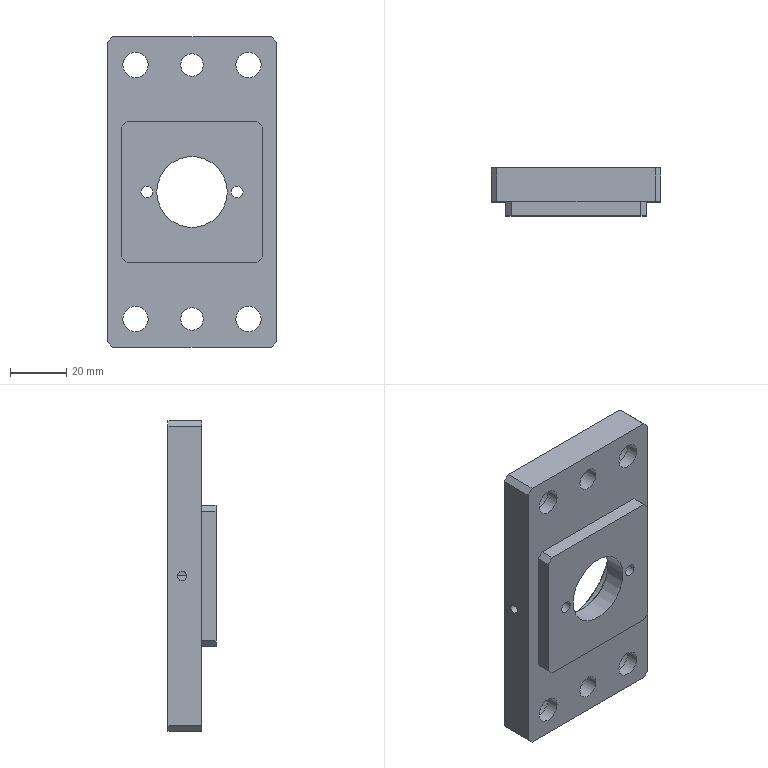Component | SolidWorks | 300-02-1 | 1 solid | 114 faces | box 60 x 17 x 110 mm | volume 65342 mm3 | plane 50 | cylinder 30 | spline 30 | cone 4 | commonest cylinder face diameters 15 x8 9 x8 8 x4 4.2 x4 3.3 x2 45 x2 25 x2 | material Cr12MoV
build123d program:
from build123d import *

# Parameters (mm, degrees)
SKETCH1_W                                          = 110
SKETCH1_H                                          = 60
BOSS_EXTRUDE1_DEPTH                                = 12
CHAMFER1_SIZE                                      = 2
SKETCH9_W                                          = 50
SKETCH9_H                                          = 50
BOSS_EXTRUDE2_DEPTH                                = 5
SKETCH2_R                                          = 12.5
CUT_EXTRUDE1_DEPTH                                 = 65.915
SKETCH5_R                                          = 22.5
CUT_EXTRUDE2_DEPTH                                 = 9
M5_TAPPED_HOLE1_D                                  = 4.2
CHAMFER2_SIZE                                      = 2
HOLE_SIZE_ACCORDING_TO_TYPE_OF_HEXAGON_D           = 9
HOLE_SIZE_ACCORDING_TO_TYPE_OF_HEXAGON_CBORE_D     = 15
HOLE_SIZE_ACCORDING_TO_TYPE_OF_HEXAGON_CBORE_DEPTH = 7.5
SIZE_MM_DOWEL_PIN_HOLE1_D                          = 8
CHAMFER3_SIZE                                      = 0.5
CUT_EXTRUDE3_DEPTH                                 = 0.2
M4_TAPPED_HOLE1_REACH                              = 84.274
M4_TAPPED_HOLE1_BORE_R                             = 1.65


with BuildPart() as part:
    # Sketch1 → Boss-Extrude1 (new body)
    with BuildSketch(Plane(origin=(0, 0, 0), x_dir=(1, 0, 0), z_dir=(0, 1, 0))):
        Rectangle(SKETCH1_W, SKETCH1_H)
    extrude(amount=BOSS_EXTRUDE1_DEPTH)

    # Chamfer1
    chamfer1_edges = [part.edges().sort_by_distance(p)[0] for p in [
        (-55, 6, -30),
        (55, 6, -30),
        (55, 6, 30),
        (-55, 6, 30),
    ]]
    chamfer(chamfer1_edges, length=CHAMFER1_SIZE)

    # Sketch9 → Boss-Extrude2 (add)
    with BuildSketch(Plane.XZ):
        Rectangle(SKETCH9_W, SKETCH9_H)
    extrude(amount=BOSS_EXTRUDE2_DEPTH)

    # Sketch2 → Cut-Extrude1 (cut, through all)
    with BuildSketch(Plane(origin=(0, 12, 0), x_dir=(1, 0, 0), z_dir=(0, 1, 0))):
        with Locations(Location((0, 0, 0), (0, 0, 270))):
            Circle(SKETCH2_R)
    extrude(amount=-CUT_EXTRUDE1_DEPTH, mode=Mode.SUBTRACT)

    # Sketch5 → Cut-Extrude2 (cut)
    with BuildSketch(Plane(origin=(0, 12, 0), x_dir=(1, 0, 0), z_dir=(0, 1, 0))):
        with Locations(Location((0, 0, 0), (0, 0, 270))):
            Circle(SKETCH5_R)
    extrude(amount=-CUT_EXTRUDE2_DEPTH, mode=Mode.SUBTRACT)

    # M5 Tapped Hole1 (through all)
    with Locations(Plane(origin=(0, 3, 0), x_dir=(1, 0, 0), z_dir=(0, 1, 0))):
        with Locations((0, -16)):
            m5_tapped_hole1 = Hole(M5_TAPPED_HOLE1_D / 2)

    # Mirror1: M5 Tapped Hole1 across plane
    add(m5_tapped_hole1.mirror(Plane.XY), mode=Mode.SUBTRACT)

    # Chamfer2
    chamfer2_edges = [part.edges().sort_by_distance(p)[0] for p in [
        (25, -2.5, -25),
        (25, -2.5, 25),
        (-25, -2.5, 25),
        (-25, -2.5, -25),
    ]]
    chamfer(chamfer2_edges, length=CHAMFER2_SIZE)

    # Hole Size _According to_ Type of Hexagon (through all)
    with Locations(Plane(origin=(0, 12, 0), x_dir=(1, 0, 0), z_dir=(0, 1, 0))):
        with Locations((45, 20), (45, -20)):
            hole_size_according_to_type_of_hexagon = CounterBoreHole(HOLE_SIZE_ACCORDING_TO_TYPE_OF_HEXAGON_D / 2, HOLE_SIZE_ACCORDING_TO_TYPE_OF_HEXAGON_CBORE_D / 2, HOLE_SIZE_ACCORDING_TO_TYPE_OF_HEXAGON_CBORE_DEPTH)

    # Size mm Dowel Pin Hole1 (through all)
    with Locations(Plane(origin=(0, 12, 0), x_dir=(1, 0, 0), z_dir=(0, 1, 0))):
        with Locations((45, 0)):
            size_mm_dowel_pin_hole1 = Hole(SIZE_MM_DOWEL_PIN_HOLE1_D / 2)

    # Mirror2: Hole Size _According to_ Type of Hexagon, Size mm Dowel Pin Hole1 across plane
    add(hole_size_according_to_type_of_hexagon.mirror(Plane(origin=(0, 0, 0), x_dir=(0, 0, 1), z_dir=(1, 0, 0))), mode=Mode.SUBTRACT)
    add(size_mm_dowel_pin_hole1.mirror(Plane(origin=(0, 0, 0), x_dir=(0, 0, 1), z_dir=(1, 0, 0))), mode=Mode.SUBTRACT)

    # Chamfer3
    chamfer3_edges = [part.edges().sort_by_distance(p)[0] for p in [
        (0, 12, -22.5),
        (0, 3, -12.5),
    ]]
    chamfer(chamfer3_edges, length=CHAMFER3_SIZE)

    # Sketch16 → Cut-Extrude3 (cut)
    # profile 1 of 4: a face of its own
    with BuildSketch(Plane(origin=(0, 12, 0), x_dir=(1, 0, 0), z_dir=(0, 1, 0))):
        with BuildLine():
            add(Edge.make_bspline(
                [(31.308, 7.917), (31.113, 7.92), (30.732, 7.925), (30.177, 7.97), (29.654, 8.039), (29.163, 8.141), (28.705, 8.274), (28.277, 8.431), (27.88, 8.619), (27.521, 8.839), (27.198, 9.078), (26.915, 9.334), (26.675, 9.604), (26.48, 9.892), (26.324, 10.191), (26.22, 10.509), (26.151, 10.84), (26.143, 11.066), (26.139, 11.181)],
                knots=[0, 0, 0, 0, 1.382, 2.69, 3.934, 5.11, 6.234, 7.304, 8.336, 9.329, 10.28, 11.171, 12.023, 12.833, 13.62, 14.403, 15.19, 16, 16, 16, 16], degree=3))
            add(Edge.make_bspline(
                [(26.139, 11.181), (26.143, 11.291), (26.15, 11.509), (26.222, 11.829), (26.329, 12.138), (26.487, 12.434), (26.689, 12.717), (26.931, 12.99), (27.22, 13.248), (27.549, 13.492), (27.914, 13.717), (28.313, 13.912), (28.74, 14.077), (29.198, 14.211), (29.684, 14.318), (30.2, 14.389), (30.744, 14.437), (31.117, 14.442), (31.308, 14.444)],
                knots=[0, 0, 0, 0, 0.783, 1.55, 2.319, 3.103, 3.922, 4.781, 5.695, 6.669, 7.689, 8.737, 9.818, 10.943, 12.122, 13.353, 14.642, 16, 16, 16, 16], degree=3))
            add(Edge.make_bspline(
                [(31.308, 14.444), (31.494, 14.441), (31.858, 14.435), (32.39, 14.395), (32.895, 14.322), (33.373, 14.227), (33.822, 14.098), (34.244, 13.942), (34.64, 13.76), (35.004, 13.548), (35.334, 13.315), (35.623, 13.063), (35.868, 12.792), (36.071, 12.505), (36.226, 12.198), (36.335, 11.874), (36.405, 11.534), (36.413, 11.3), (36.417, 11.181)],
                knots=[0, 0, 0, 0, 1.325, 2.592, 3.8, 4.958, 6.063, 7.129, 8.158, 9.165, 10.126, 11.032, 11.894, 12.723, 13.533, 14.333, 15.153, 16, 16, 16, 16], degree=3))
            add(Edge.make_bspline(
                [(36.417, 11.181), (36.412, 11.057), (36.403, 10.815), (36.332, 10.462), (36.213, 10.131), (36.05, 9.818), (35.833, 9.53), (35.575, 9.258), (35.268, 9.008), (34.918, 8.783), (34.536, 8.582), (34.131, 8.404), (33.709, 8.25), (33.265, 8.131), (32.803, 8.034), (32.322, 7.966), (31.821, 7.923), (31.481, 7.919), (31.308, 7.917)],
                knots=[0, 0, 0, 0, 0.8798, 1.727, 2.556, 3.385, 4.238, 5.122, 6.058, 7.055, 8.09, 9.139, 10.205, 11.297, 12.415, 13.574, 14.765, 16, 16, 16, 16], degree=3))
        make_face()
        with BuildLine():
            add(Edge.make_bspline(
                [(31.336, 13.333), (31.135, 13.332), (30.745, 13.33), (30.182, 13.298), (29.662, 13.252), (29.184, 13.188), (28.749, 13.102), (28.357, 12.997), (28.006, 12.874), (27.698, 12.73), (27.431, 12.571), (27.198, 12.404), (27.001, 12.226), (26.837, 12.039), (26.712, 11.838), (26.622, 11.628), (26.565, 11.408), (26.559, 11.257), (26.556, 11.181)],
                knots=[0, 0, 0, 0, 1.687, 3.255, 4.711, 6.048, 7.281, 8.414, 9.441, 10.382, 11.246, 12.038, 12.774, 13.46, 14.109, 14.74, 15.363, 16, 16, 16, 16], degree=3))
            add(Edge.make_bspline(
                [(26.556, 11.181), (26.559, 11.1), (26.566, 10.942), (26.617, 10.71), (26.702, 10.492), (26.822, 10.287), (26.975, 10.095), (27.165, 9.919), (27.385, 9.754), (27.64, 9.6), (27.937, 9.462), (28.282, 9.347), (28.674, 9.248), (29.113, 9.166), (29.601, 9.105), (30.136, 9.061), (30.72, 9.032), (31.126, 9.029), (31.336, 9.028)],
                knots=[0, 0, 0, 0, 0.6675, 1.312, 1.956, 2.601, 3.276, 3.984, 4.742, 5.555, 6.449, 7.45, 8.564, 9.797, 11.152, 12.639, 14.254, 16, 16, 16, 16], degree=3))
            add(Edge.make_bspline(
                [(31.336, 9.028), (31.507, 9.03), (31.84, 9.034), (32.327, 9.054), (32.788, 9.094), (33.224, 9.147), (33.634, 9.217), (34.019, 9.3), (34.378, 9.403), (34.712, 9.515), (35.014, 9.648), (35.278, 9.801), (35.5, 9.979), (35.683, 10.178), (35.827, 10.398), (35.927, 10.641), (35.99, 10.904), (35.997, 11.087), (36, 11.181)],
                knots=[0, 0, 0, 0, 1.442, 2.813, 4.113, 5.351, 6.522, 7.63, 8.678, 9.673, 10.603, 11.455, 12.247, 12.999, 13.728, 14.457, 15.21, 16, 16, 16, 16], degree=3))
            add(Edge.make_bspline(
                [(36, 11.181), (35.997, 11.261), (35.992, 11.42), (35.931, 11.651), (35.841, 11.87), (35.711, 12.076), (35.545, 12.267), (35.34, 12.443), (35.102, 12.609), (34.827, 12.76), (34.516, 12.897), (34.169, 13.013), (33.786, 13.112), (33.366, 13.194), (32.909, 13.256), (32.417, 13.3), (31.889, 13.329), (31.524, 13.332), (31.336, 13.333)],
                knots=[0, 0, 0, 0, 0.6848, 1.35, 2.018, 2.692, 3.408, 4.166, 4.984, 5.871, 6.833, 7.866, 8.985, 10.195, 11.5, 12.903, 14.4, 16, 16, 16, 16], degree=3))
        make_face(mode=Mode.SUBTRACT)
    # profile 2 of 4: a face of its own
    with BuildSketch(Plane(origin=(0, 12, 0), x_dir=(1, 0, 0), z_dir=(0, 1, 0))):
        with BuildLine():
            Line((31, 5.278), (27.159, 5.278))
            add(Edge.make_bspline(
                [(27.159, 5.278), (27.123, 5.276), (27.053, 5.273), (26.956, 5.25), (26.874, 5.208), (26.807, 5.15), (26.757, 5.079), (26.72, 4.998), (26.697, 4.906), (26.695, 4.842), (26.694, 4.809)],
                knots=[0, 0, 0, 0, 1.162, 2.213, 3.177, 4.097, 5.01, 5.954, 6.932, 8, 8, 8, 8], degree=3))
            Line((26.694, 4.809), (26.694, 4.444))
            Line((26.694, 4.444), (26.278, 4.444))
            Line((26.278, 4.444), (26.278, 7.083))
            Line((26.278, 7.083), (26.694, 7.083))
            Line((26.694, 7.083), (26.694, 6.719))
            add(Edge.make_bspline(
                [(26.694, 6.719), (26.695, 6.679), (26.697, 6.604), (26.717, 6.501), (26.755, 6.418), (26.806, 6.351), (26.875, 6.305), (26.957, 6.273), (27.052, 6.253), (27.12, 6.251), (27.157, 6.25)],
                knots=[0, 0, 0, 0, 1.254, 2.348, 3.275, 4.117, 4.951, 5.86, 6.86, 8, 8, 8, 8], degree=3))
            Line((27.157, 6.25), (35.399, 6.25))
            add(Edge.make_bspline(
                [(35.399, 6.25), (35.435, 6.251), (35.504, 6.253), (35.6, 6.274), (35.681, 6.31), (35.749, 6.358), (35.801, 6.428), (35.838, 6.517), (35.859, 6.627), (35.86, 6.706), (35.861, 6.749)],
                knots=[0, 0, 0, 0, 1.103, 2.098, 2.965, 3.785, 4.618, 5.575, 6.699, 8, 8, 8, 8], degree=3))
            Line((35.861, 6.749), (35.861, 7.083))
            Line((35.861, 7.083), (36.278, 7.083))
            Line((36.278, 7.083), (36.278, 3.613))
            add(Edge.make_bspline(
                [(36.278, 3.613), (36.276, 3.495), (36.273, 3.263), (36.237, 2.927), (36.181, 2.611), (36.103, 2.316), (36.002, 2.041), (35.875, 1.788), (35.727, 1.556), (35.557, 1.348), (35.372, 1.161), (35.17, 1), (34.96, 0.862), (34.735, 0.7515), (34.501, 0.6602), (34.252, 0.6015), (33.992, 0.5631), (33.816, 0.5581), (33.726, 0.5556)],
                knots=[0, 0, 0, 0, 1.27, 2.476, 3.616, 4.697, 5.738, 6.742, 7.716, 8.674, 9.615, 10.529, 11.424, 12.306, 13.2, 14.109, 15.039, 16, 16, 16, 16], degree=3))
            add(Edge.make_bspline(
                [(33.726, 0.5556), (33.618, 0.5576), (33.407, 0.5616), (33.103, 0.6056), (32.816, 0.667), (32.552, 0.766), (32.305, 0.8832), (32.08, 1.033), (31.874, 1.208), (31.69, 1.408), (31.529, 1.627), (31.388, 1.857), (31.267, 2.097), (31.169, 2.348), (31.094, 2.609), (31.039, 2.879), (31.006, 3.16), (31.002, 3.351), (31, 3.448)],
                knots=[0, 0, 0, 0, 1.156, 2.252, 3.294, 4.292, 5.267, 6.224, 7.181, 8.152, 9.128, 10.092, 11.045, 12.003, 12.972, 13.953, 14.96, 16, 16, 16, 16], degree=3))
            Line((31, 3.448), (31, 5.278))
        make_face()
        with BuildLine():
            add(Edge.make_bspline(
                [(31.417, 3.845), (31.418, 3.775), (31.422, 3.634), (31.446, 3.428), (31.486, 3.227), (31.539, 3.033), (31.612, 2.846), (31.699, 2.665), (31.801, 2.489), (31.92, 2.321), (32.058, 2.166), (32.22, 2.03), (32.407, 1.917), (32.616, 1.826), (32.847, 1.755), (33.1, 1.703), (33.376, 1.673), (33.568, 1.669), (33.667, 1.667)],
                knots=[0, 0, 0, 0, 0.9555, 1.887, 2.8, 3.701, 4.598, 5.496, 6.408, 7.33, 8.261, 9.202, 10.172, 11.184, 12.266, 13.42, 14.664, 16, 16, 16, 16], degree=3))
            add(Edge.make_bspline(
                [(33.667, 1.667), (33.758, 1.668), (33.933, 1.671), (34.187, 1.698), (34.423, 1.737), (34.64, 1.799), (34.84, 1.875), (35.021, 1.968), (35.184, 2.08), (35.329, 2.209), (35.456, 2.358), (35.564, 2.527), (35.659, 2.715), (35.731, 2.925), (35.789, 3.156), (35.833, 3.406), (35.856, 3.677), (35.859, 3.864), (35.861, 3.961)],
                knots=[0, 0, 0, 0, 1.184, 2.298, 3.337, 4.32, 5.244, 6.129, 6.98, 7.819, 8.665, 9.535, 10.445, 11.41, 12.446, 13.551, 14.73, 16, 16, 16, 16], degree=3))
            Line((35.861, 3.961), (35.861, 4.761))
            add(Edge.make_bspline(
                [(35.861, 4.761), (35.86, 4.798), (35.859, 4.869), (35.835, 4.969), (35.802, 5.059), (35.751, 5.136), (35.688, 5.201), (35.607, 5.247), (35.513, 5.273), (35.447, 5.276), (35.412, 5.278)],
                knots=[0, 0, 0, 0, 1.143, 2.174, 3.159, 4.096, 5.013, 5.945, 6.922, 8, 8, 8, 8], degree=3))
            Line((35.412, 5.278), (31.417, 5.278))
            Line((31.417, 5.278), (31.417, 3.845))
        make_face(mode=Mode.SUBTRACT)
    # profile 3 of 4: a face of its own
    with BuildSketch(Plane(origin=(0, 12, 0), x_dir=(1, 0, 0), z_dir=(0, 1, 0))):
        with BuildLine():
            add(Edge.make_bspline(
                [(35.868, -6.667), (35.702, -6.561), (35.375, -6.352), (34.881, -6.052), (34.39, -5.768), (33.901, -5.501), (33.415, -5.252), (32.932, -5.018), (32.451, -4.802), (31.976, -4.6), (31.509, -4.42), (31.056, -4.264), (30.619, -4.131), (30.197, -4.021), (29.79, -3.937), (29.399, -3.875), (29.024, -3.839), (28.779, -3.833), (28.658, -3.83)],
                knots=[0, 0, 0, 0, 1.201, 2.378, 3.539, 4.675, 5.79, 6.882, 7.961, 9.019, 10.044, 11.023, 11.954, 12.841, 13.692, 14.499, 15.264, 16, 16, 16, 16], degree=3))
            add(Edge.make_bspline(
                [(28.658, -3.83), (28.615, -3.831), (28.52, -3.833), (28.364, -3.836), (28.182, -3.849), (27.977, -3.861), (27.749, -3.875), (27.503, -3.883), (27.237, -3.887), (27.054, -3.888), (26.959, -3.889)],
                knots=[0, 0, 0, 0, 0.6126, 1.348, 2.197, 3.179, 4.252, 5.417, 6.663, 8, 8, 8, 8], degree=3))
            add(Edge.make_bspline(
                [(26.959, -3.889), (26.887, -3.888), (26.754, -3.885), (26.574, -3.859), (26.428, -3.821), (26.313, -3.762), (26.233, -3.675), (26.176, -3.568), (26.144, -3.437), (26.141, -3.343), (26.139, -3.292)],
                knots=[0, 0, 0, 0, 1.474, 2.695, 3.706, 4.53, 5.28, 6.084, 6.966, 8, 8, 8, 8], degree=3))
            add(Edge.make_bspline(
                [(26.139, -3.292), (26.141, -3.248), (26.145, -3.161), (26.188, -3.038), (26.251, -2.925), (26.345, -2.823), (26.472, -2.735), (26.642, -2.68), (26.848, -2.642), (26.999, -2.64), (27.081, -2.639)],
                knots=[0, 0, 0, 0, 0.8206, 1.595, 2.381, 3.215, 4.14, 5.207, 6.486, 8, 8, 8, 8], degree=3))
            add(Edge.make_bspline(
                [(27.081, -2.639), (27.177, -2.641), (27.375, -2.645), (27.68, -2.667), (28.001, -2.708), (28.339, -2.761), (28.693, -2.835), (29.065, -2.918), (29.452, -3.021), (29.788, -3.117), (30.072, -3.209), (30.306, -3.288), (30.556, -3.386), (30.824, -3.494), (31.112, -3.613), (31.417, -3.748), (31.74, -3.896), (32.082, -4.054), (32.439, -4.228), (32.815, -4.415), (33.209, -4.614), (33.621, -4.827), (34.052, -5.051), (34.5, -5.289), (34.967, -5.541), (35.283, -5.714), (35.444, -5.803)],
                knots=[0, 0, 0, 0, 0.7676, 1.577, 2.437, 3.349, 4.308, 5.32, 6.388, 7.505, 8.105, 8.764, 9.474, 10.245, 11.07, 11.959, 12.904, 13.902, 14.96, 16.075, 17.251, 18.485, 19.772, 21.124, 22.534, 24, 24, 24, 24], degree=3))
            Line((35.444, -5.803), (35.444, -2.873))
            add(Edge.make_bspline(
                [(35.444, -2.873), (35.44, -2.772), (35.431, -2.578), (35.351, -2.302), (35.218, -2.061), (35.029, -1.853), (34.789, -1.676), (34.498, -1.527), (34.157, -1.403), (33.909, -1.347), (33.778, -1.317)],
                knots=[0, 0, 0, 0, 0.9673, 1.863, 2.719, 3.593, 4.529, 5.562, 6.714, 8, 8, 8, 8], degree=3))
            Line((33.778, -1.317), (33.836, -0.9722))
            Line((33.836, -0.9722), (36.278, -1.382))
            Line((36.278, -1.382), (36.278, -6.667))
            Line((36.278, -6.667), (35.868, -6.667))
        make_face()
    # profile 4 of 4: a face of its own
    with BuildSketch(Plane(origin=(0, 12, 0), x_dir=(1, 0, 0), z_dir=(0, 1, 0))):
        with BuildLine():
            add(Edge.make_bspline(
                [(26.139, -11.209), (26.143, -11.104), (26.151, -10.898), (26.217, -10.595), (26.321, -10.304), (26.473, -10.029), (26.665, -9.765), (26.899, -9.515), (27.175, -9.278), (27.492, -9.056), (27.847, -8.851), (28.24, -8.677), (28.667, -8.527), (29.128, -8.404), (29.624, -8.309), (30.155, -8.243), (30.72, -8.201), (31.108, -8.197), (31.308, -8.194)],
                knots=[0, 0, 0, 0, 0.7573, 1.497, 2.234, 2.992, 3.77, 4.594, 5.468, 6.406, 7.397, 8.433, 9.523, 10.675, 11.893, 13.184, 14.552, 16, 16, 16, 16], degree=3))
            add(Edge.make_bspline(
                [(31.308, -8.194), (31.494, -8.197), (31.858, -8.202), (32.39, -8.24), (32.894, -8.309), (33.372, -8.397), (33.821, -8.518), (34.244, -8.659), (34.638, -8.832), (35.003, -9.028), (35.333, -9.243), (35.621, -9.478), (35.868, -9.726), (36.069, -9.992), (36.227, -10.273), (36.334, -10.572), (36.405, -10.885), (36.413, -11.1), (36.417, -11.209)],
                knots=[0, 0, 0, 0, 1.361, 2.662, 3.902, 5.088, 6.217, 7.302, 8.348, 9.364, 10.328, 11.231, 12.077, 12.887, 13.662, 14.429, 15.204, 16, 16, 16, 16], degree=3))
            add(Edge.make_bspline(
                [(36.417, -11.209), (36.412, -11.313), (36.404, -11.519), (36.339, -11.821), (36.232, -12.109), (36.082, -12.383), (35.892, -12.644), (35.655, -12.887), (35.379, -13.12), (35.062, -13.335), (34.709, -13.533), (34.319, -13.701), (33.898, -13.848), (33.442, -13.962), (32.956, -14.057), (32.436, -14.12), (31.883, -14.16), (31.504, -14.164), (31.308, -14.167)],
                knots=[0, 0, 0, 0, 0.7676, 1.512, 2.261, 3.018, 3.802, 4.626, 5.509, 6.45, 7.443, 8.476, 9.568, 10.716, 11.929, 13.21, 14.564, 16, 16, 16, 16], degree=3))
            add(Edge.make_bspline(
                [(31.308, -14.167), (31.113, -14.164), (30.732, -14.16), (30.178, -14.12), (29.655, -14.057), (29.165, -13.962), (28.705, -13.848), (28.279, -13.7), (27.882, -13.534), (27.522, -13.335), (27.198, -13.12), (26.918, -12.887), (26.675, -12.645), (26.481, -12.383), (26.325, -12.11), (26.22, -11.821), (26.151, -11.519), (26.143, -11.313), (26.139, -11.209)],
                knots=[0, 0, 0, 0, 1.426, 2.775, 4.057, 5.266, 6.416, 7.509, 8.554, 9.553, 10.501, 11.385, 12.214, 12.998, 13.755, 14.498, 15.238, 16, 16, 16, 16], degree=3))
        make_face()
        with BuildLine():
            add(Edge.make_bspline(
                [(36, -11.209), (35.996, -11.142), (35.989, -11.009), (35.925, -10.816), (35.822, -10.632), (35.681, -10.457), (35.497, -10.293), (35.277, -10.133), (35.013, -9.988), (34.716, -9.847), (34.384, -9.721), (34.024, -9.607), (33.637, -9.516), (33.223, -9.436), (32.783, -9.38), (32.315, -9.336), (31.821, -9.31), (31.482, -9.307), (31.308, -9.306)],
                knots=[0, 0, 0, 0, 0.5824, 1.171, 1.775, 2.427, 3.144, 3.938, 4.816, 5.788, 6.832, 7.94, 9.106, 10.338, 11.642, 13.017, 14.471, 16, 16, 16, 16], degree=3))
            add(Edge.make_bspline(
                [(31.308, -9.306), (31.125, -9.307), (30.77, -9.31), (30.252, -9.336), (29.766, -9.38), (29.312, -9.436), (28.89, -9.516), (28.498, -9.607), (28.138, -9.72), (27.81, -9.847), (27.518, -9.988), (27.261, -10.133), (27.047, -10.293), (26.868, -10.457), (26.729, -10.632), (26.628, -10.816), (26.567, -11.01), (26.559, -11.143), (26.556, -11.209)],
                knots=[0, 0, 0, 0, 1.592, 3.091, 4.505, 5.831, 7.072, 8.236, 9.33, 10.35, 11.293, 12.144, 12.913, 13.611, 14.252, 14.846, 15.425, 16, 16, 16, 16], degree=3))
            add(Edge.make_bspline(
                [(26.556, -11.209), (26.559, -11.279), (26.567, -11.419), (26.628, -11.622), (26.728, -11.812), (26.867, -11.99), (27.046, -12.153), (27.262, -12.306), (27.517, -12.446), (27.811, -12.572), (28.138, -12.687), (28.499, -12.785), (28.89, -12.87), (29.313, -12.936), (29.766, -12.99), (30.252, -13.029), (30.77, -13.05), (31.125, -13.054), (31.308, -13.056)],
                knots=[0, 0, 0, 0, 0.6126, 1.216, 1.826, 2.471, 3.165, 3.923, 4.764, 5.691, 6.697, 7.78, 8.939, 10.174, 11.498, 12.911, 14.409, 16, 16, 16, 16], degree=3))
            add(Edge.make_bspline(
                [(31.308, -13.056), (31.482, -13.055), (31.821, -13.052), (32.315, -13.031), (32.782, -12.993), (33.223, -12.945), (33.636, -12.879), (34.023, -12.802), (34.383, -12.71), (34.715, -12.602), (35.014, -12.48), (35.277, -12.345), (35.498, -12.192), (35.682, -12.027), (35.824, -11.844), (35.926, -11.646), (35.99, -11.432), (35.997, -11.284), (36, -11.209)],
                knots=[0, 0, 0, 0, 1.521, 2.967, 4.333, 5.628, 6.847, 7.998, 9.084, 10.104, 11.05, 11.909, 12.688, 13.401, 14.065, 14.705, 15.345, 16, 16, 16, 16], degree=3))
        make_face(mode=Mode.SUBTRACT)
    extrude(amount=-CUT_EXTRUDE3_DEPTH, mode=Mode.SUBTRACT)

    # M4 Tapped Hole1 bore → M4 Tapped Hole1 (cut, up to next)
    with BuildSketch(Plane(origin=(0, 0, -30), x_dir=(1, 0, 0), z_dir=(0, 0, -1)), mode=Mode.PRIVATE) as m4_tapped_hole1_sk1:
        with Locations((0, -7)):
            Circle(M4_TAPPED_HOLE1_BORE_R)
    m4_tapped_hole1_tool1 = extrude(m4_tapped_hole1_sk1.sketch, amount=-M4_TAPPED_HOLE1_REACH, mode=Mode.PRIVATE) & part.part
    add(m4_tapped_hole1_tool1.solids().sort_by_distance((0, 7, -30))[0], mode=Mode.SUBTRACT)


solid = part.part

# Placed as in the assembly
solid = solid.moved(Location((230, 153, 0), (0, 90, 0)))